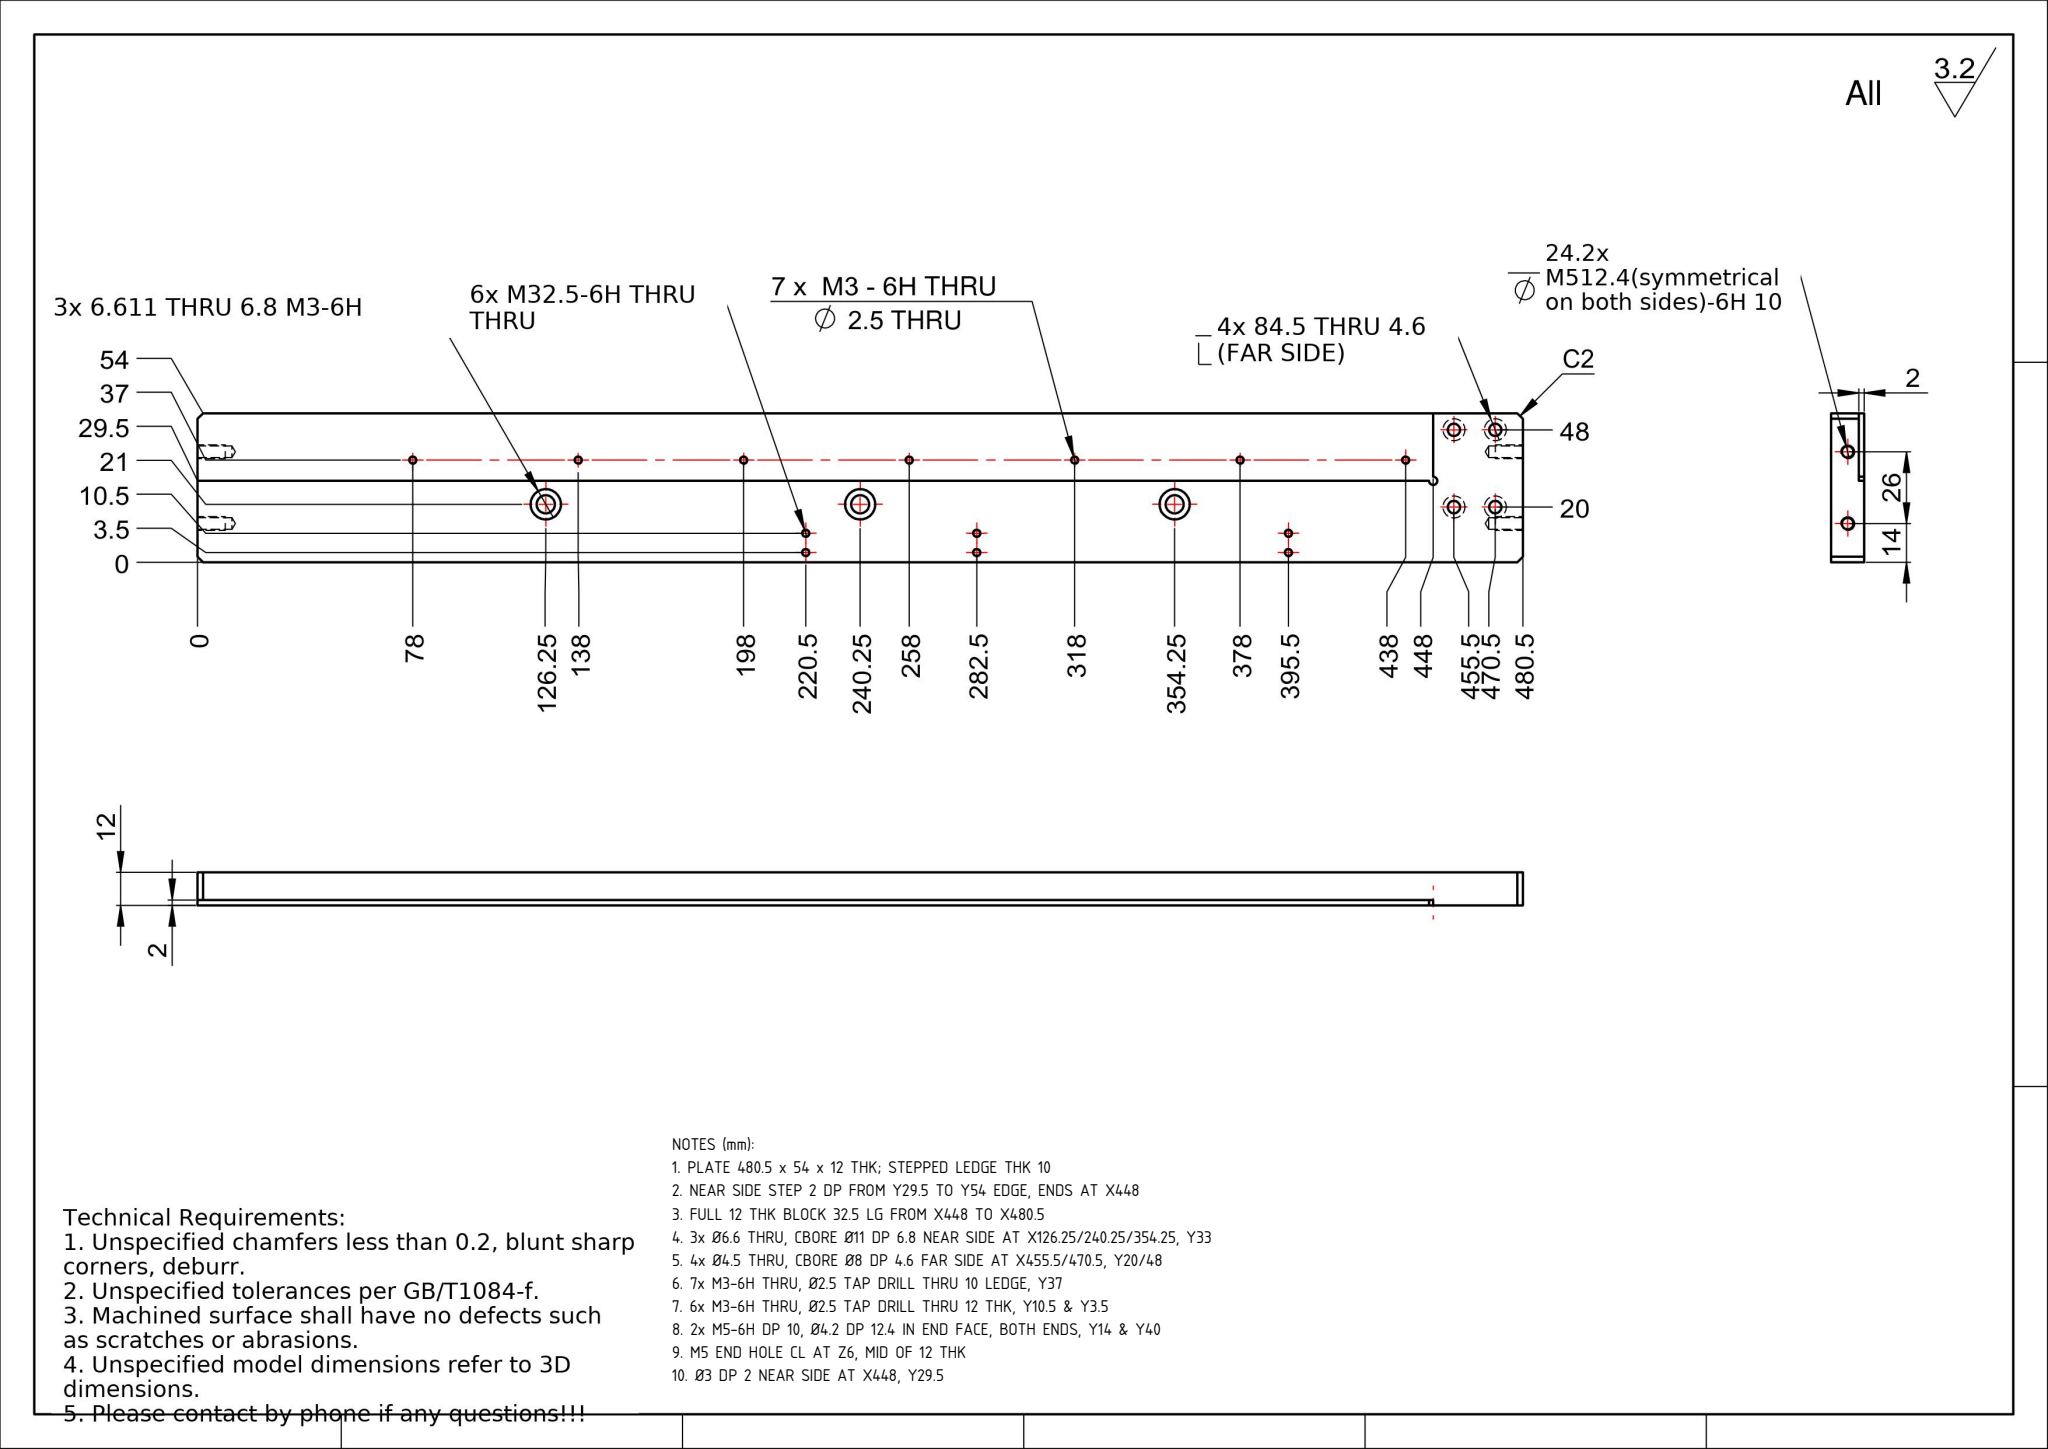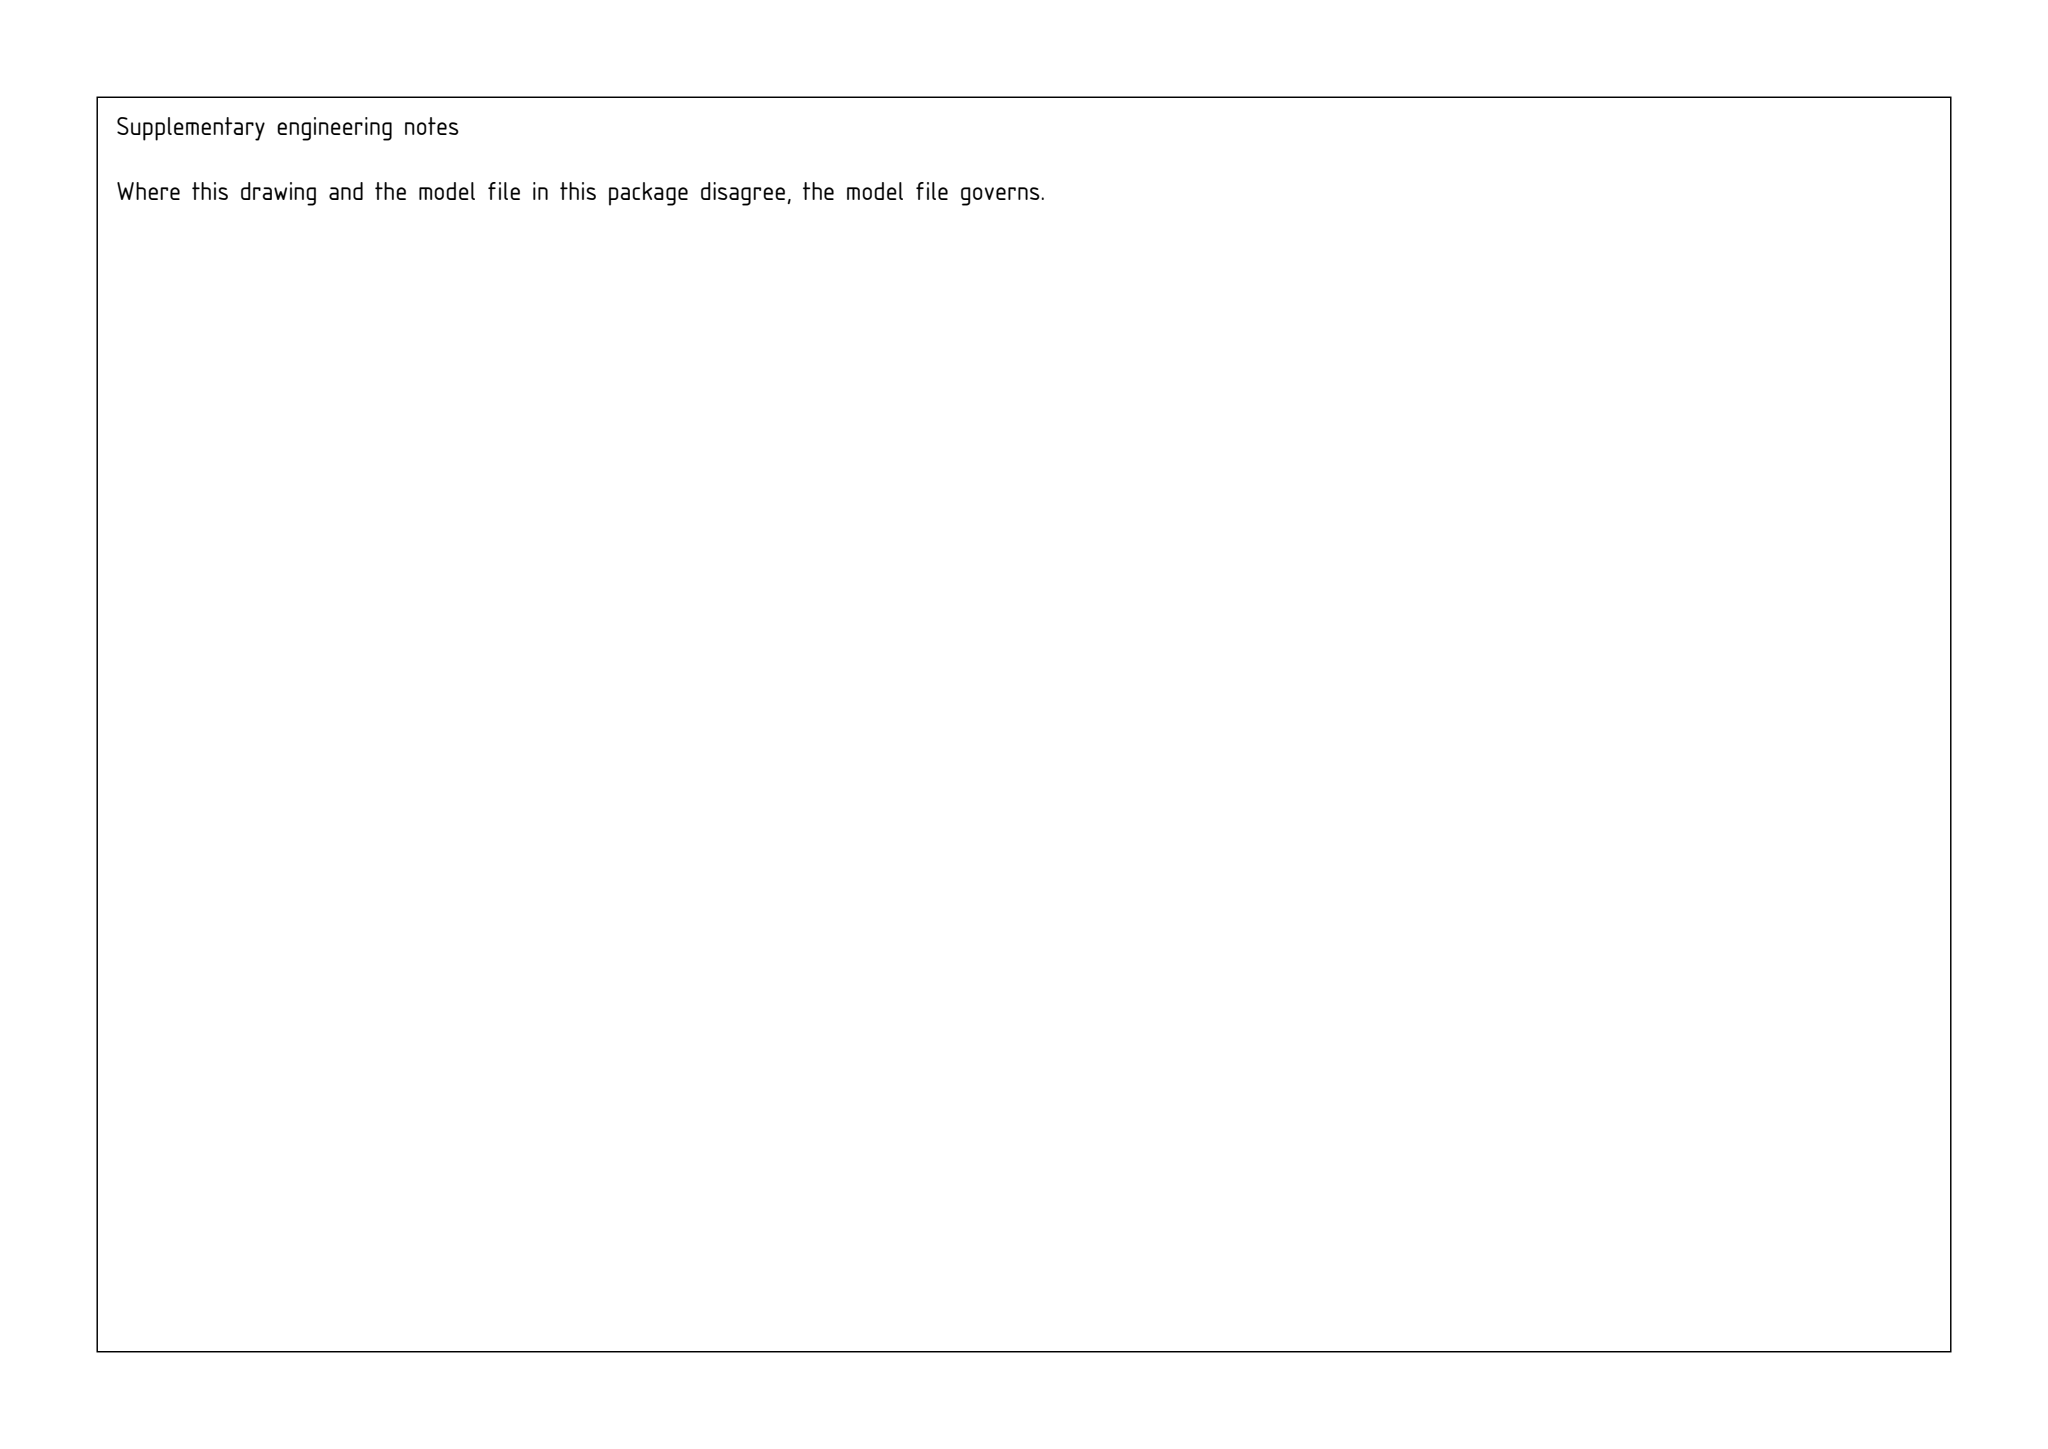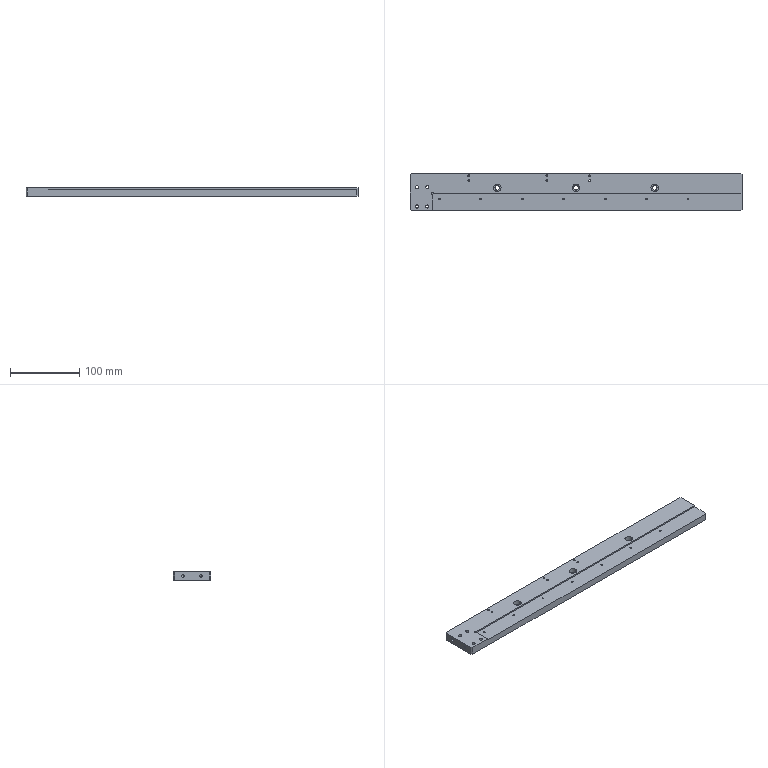Part | SolidWorks | mm | 1 solid | 91 faces | box 480.5 x 54 x 12 mm | volume 284034 mm3 | cylinder 63 | plane 20 | cone 8 | commonest cylinder face diameters 2.5 x26 8 x8 4.5 x8 4.2 x8 11 x6 6.6 x6 3 x1
Drawing notes:
PLATE 480.5 x 54 x 12 THK; STEPPED LEDGE THK 10 | from the solid: bbox 480.5x54x12; z plane at 10.0; Ø2.5 ledge holes L10
NEAR SIDE STEP 2 DP FROM Y29.5 TO Y54 EDGE, ENDS AT X448 | from the solid: z planes 10.0/12.0 (12-10=2); y plane 24.5 = dwg 29.5; x plane 32.5 = dwg X448
FULL 12 THK BLOCK 32.5 LG FROM X448 TO X480.5 | from the solid: axis_plane x=32.5 step wall with bbox x=480.5
3x Ø6.6 THRU, CBORE Ø11 DP 6.8 NEAR SIDE AT X126.25/240.25/354.25, Y33 | from the solid: Ø6.6 L5.2 + Ø11 L6.8 coaxial at x=126.25/240.25/354.25, y=33; 5.2+6.8=12
4x Ø4.5 THRU, CBORE Ø8 DP 4.6 FAR SIDE AT X455.5/470.5, Y20/48 | from the solid: Ø4.5 L7.4 + Ø8 L4.6 at x=10,25 (dwg 470.5,455.5), y=6,34 (dwg 48,20); 7.4+4.6=12
7x M3-6H THRU, Ø2.5 TAP DRILL THRU 10 LEDGE, Y37 | from the solid: Ø2.5 z-holes L10 at x=42.5..402.5 step 60 (dwg 78..438), y=17 (dwg 37)
6x M3-6H THRU, Ø2.5 TAP DRILL THRU 12 THK, Y10.5 & Y3.5 | from the solid: Ø2.5 z-holes L12 at x=85,198,260 (dwg 395.5,282.5,220.5), y=43.5/50.5
2x M5-6H DP 10, Ø4.2 DP 12.4 IN END FACE, BOTH ENDS, Y14 & Y40 | from the solid: Ø4.2 x-axis cyls L12.4 at y=14 & 40, 118° drill points, symmetric both ends
M5 END HOLE CL AT Z6, MID OF 12 THK | from the solid: Ø4.2 x-axis cyls at z=6.0; bbox z=12.0
Ø3 DP 2 NEAR SIDE AT X448, Y29.5 | from the solid: Ø3.0 z-cyl L2.0 at x=32.5 (dwg 448), y=24.5 (dwg 29.5)
build123d program:
from build123d import *

# Parameters (mm, degrees)
SKETCH1_W                                            = 480.5
SKETCH1_H                                            = 54
BOSS_EXTRUDE1_DEPTH                                  = 6
SKETCH2_W                                            = 448
SKETCH2_H                                            = 24.5
CUT_EXTRUDE1_DEPTH                                   = 2
M3_TAPPED_HOLE2_D                                    = 2.5
LPATTERN1_COUNT                                      = 7
LPATTERN1_PITCH                                      = 60
M5_TAPPED_HOLE1_D                                    = 4.2
M5_TAPPED_HOLE1_DEPTH                                = 12.4
M5_TAPPED_HOLE1_TIP                                  = 1.262
M5_TAPPED_HOLE2_D                                    = 4.2
M5_TAPPED_HOLE2_DEPTH                                = 12.4
M5_TAPPED_HOLE2_TIP                                  = 1.262
M3_TAPPED_HOLE1_D                                    = 2.5
HOLE_SIZE_ACCORDING_TO_THE_TYPE_OF_HEXAG_D           = 4.5
HOLE_SIZE_ACCORDING_TO_THE_TYPE_OF_HEXAG_CBORE_D     = 8
HOLE_SIZE_ACCORDING_TO_THE_TYPE_OF_HEXAG_CBORE_DEPTH = 4.6
HOLE_SIZE_ACCORDING_TO_THE_TYPE_OF_HE_D              = 6.6
HOLE_SIZE_ACCORDING_TO_THE_TYPE_OF_HE_CBORE_D        = 11
HOLE_SIZE_ACCORDING_TO_THE_TYPE_OF_HE_CBORE_DEPTH    = 6.8
SKETCH23_R                                           = 1.5
CUT_EXTRUDE4_DEPTH                                   = 2
CHAMFER1_SIZE                                        = 2


with BuildPart() as part:
    # Sketch1 → Boss-Extrude1 (new, symmetric)
    with BuildSketch(Plane.XY):
        Rectangle(SKETCH1_W, SKETCH1_H)
    extrude(amount=BOSS_EXTRUDE1_DEPTH, both=True)

    # Sketch2 → Cut-Extrude1 (cut)
    with BuildSketch(Plane.XY.offset(6)):
        with Locations((16.25, -14.75)):
            Rectangle(SKETCH2_W, SKETCH2_H)
    extrude(amount=-CUT_EXTRUDE1_DEPTH, mode=Mode.SUBTRACT)

    # M3 Tapped Hole2 (through all)
    with Locations(Plane.XY.offset(4)):
        with Locations((162.25, -10)):
            m3_tapped_hole2 = Hole(M3_TAPPED_HOLE2_D / 2)

    # LPattern1: M3 Tapped Hole2 ×7
    with Locations(*[(-i * LPATTERN1_PITCH, 0, 0) for i in range(1, LPATTERN1_COUNT)]):
        add(m3_tapped_hole2, mode=Mode.SUBTRACT)

    # M5 Tapped Hole1
    with Locations(Plane(origin=(240.25, 0, 0), x_dir=(0, 0, -1), z_dir=(1, 0, 0))):
        with Locations((0, 13), (0, -13)):
            Hole(M5_TAPPED_HOLE1_D / 2, depth=M5_TAPPED_HOLE1_DEPTH)
            with Locations((0, 0, -(M5_TAPPED_HOLE1_DEPTH + M5_TAPPED_HOLE1_TIP / 2))):  # 118° drill point
                Cone(0, M5_TAPPED_HOLE1_D / 2, M5_TAPPED_HOLE1_TIP, mode=Mode.SUBTRACT)

    # M5 Tapped Hole2
    with Locations(Plane.ZY.offset(240.25)):
        with Locations((0, 13), (0, -13)):
            Hole(M5_TAPPED_HOLE2_D / 2, depth=M5_TAPPED_HOLE2_DEPTH)
            with Locations((0, 0, -(M5_TAPPED_HOLE2_DEPTH + M5_TAPPED_HOLE2_TIP / 2))):  # 118° drill point
                Cone(0, M5_TAPPED_HOLE2_D / 2, M5_TAPPED_HOLE2_TIP, mode=Mode.SUBTRACT)

    # M3 Tapped Hole1 (through all)
    with Locations(Plane.XY.offset(6)):
        with Locations((-42.25, 23.5), (-42.25, 16.5), (-155.25, 23.5), (-155.25, 16.5), (19.75, 23.5), (19.75, 16.5)):
            Hole(M3_TAPPED_HOLE1_D / 2)

    # Hole Size according to the type of hexag (through all)
    with Locations(Plane(origin=(0, 0, -6), x_dir=(-1, 0, 0), z_dir=(0, 0, -1))):
        with Locations((230.25, -21), (215.25, -21), (230.25, 7), (215.25, 7)):
            CounterBoreHole(HOLE_SIZE_ACCORDING_TO_THE_TYPE_OF_HEXAG_D / 2, HOLE_SIZE_ACCORDING_TO_THE_TYPE_OF_HEXAG_CBORE_D / 2, HOLE_SIZE_ACCORDING_TO_THE_TYPE_OF_HEXAG_CBORE_DEPTH)

    # Hole Size _ according to_ the type of he (through all)
    with Locations(Plane.XY.offset(6)):
        with Locations((114, 6), (0, 6), (-114, 6)):
            CounterBoreHole(HOLE_SIZE_ACCORDING_TO_THE_TYPE_OF_HE_D / 2, HOLE_SIZE_ACCORDING_TO_THE_TYPE_OF_HE_CBORE_D / 2, HOLE_SIZE_ACCORDING_TO_THE_TYPE_OF_HE_CBORE_DEPTH)

    # Sketch23 → Cut-Extrude4 (cut)
    with BuildSketch(Plane.XY.offset(6)):
        with Locations((-207.75, -2.5)):
            Circle(SKETCH23_R)
    extrude(amount=-CUT_EXTRUDE4_DEPTH, mode=Mode.SUBTRACT)

    # Chamfer1
    chamfer1_edges = [part.edges().sort_by_distance(p)[0] for p in [
        (240.25, -27, -1),
        (-240.25, -27, 0),
        (-240.25, 27, 0),
        (240.25, 27, 0),
    ]]
    chamfer(chamfer1_edges, length=CHAMFER1_SIZE)


solid = part.part